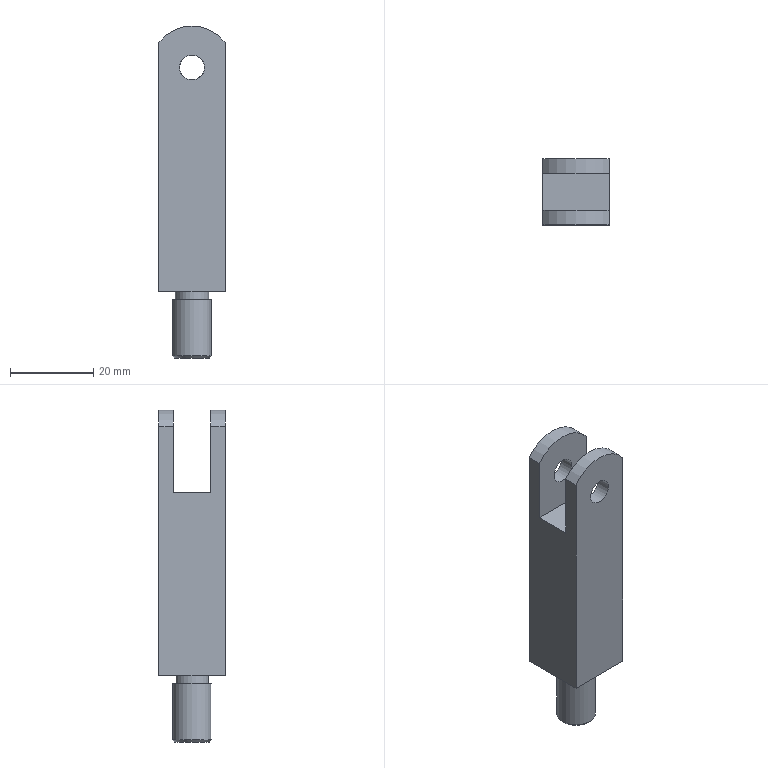Component | NX | SUPPORT | 1 solid | 17 faces | volume 14241 mm3 | plane 10 | cylinder 6 | cone 1 | commonest cylinder face diameters 20 x2 6 x2 9.373 x1 8 x1